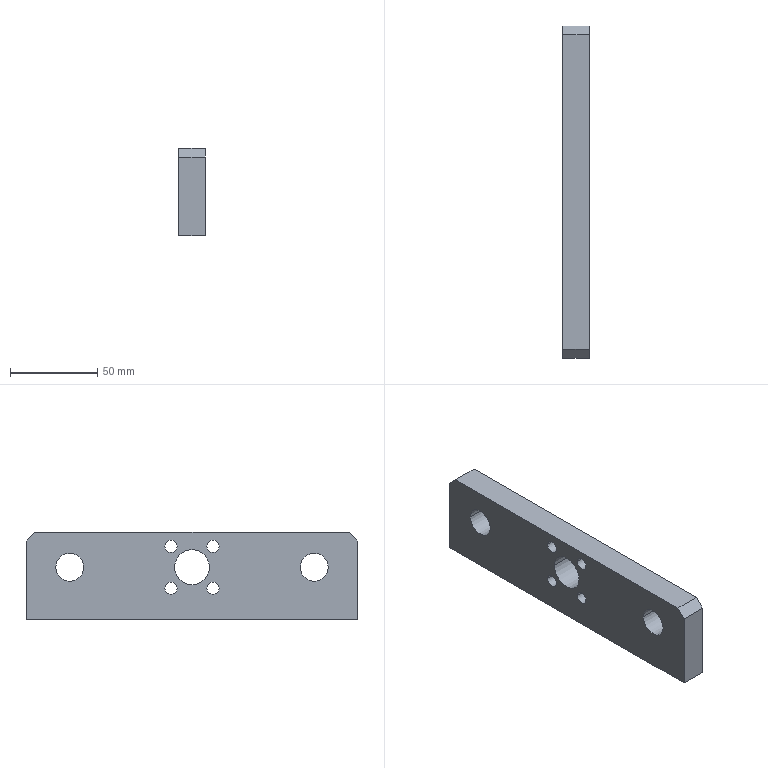Component | SolidWorks | DoubleFilmTransport-1_SupportPlate-1 | 1 solid | 46 faces | box 15 x 190 x 50 mm | volume 124028 mm3 | cylinder 26 | plane 12 | cone 8 | commonest cylinder face diameters 11 x8 7 x8 8.5 x4 16 x4 20 x2
build123d program:
from build123d import *

# Parameters (mm, degrees)
SKETCH1_W                                            = 190
SKETCH1_H                                            = 50
BOSS_EXTRUDE1_DEPTH                                  = 15
F_20_0_20_DIAMETER_HOLE1_D                           = 20
F_16_0_16_DIAMETER_HOLE1_D                           = 16
CYLINDRICAL_COUNTERSUNK_HOLE_1_FOR_M6_HE_D           = 7
CYLINDRICAL_COUNTERSUNK_HOLE_1_FOR_M6_HE_CBORE_D     = 11
CYLINDRICAL_COUNTERSUNK_HOLE_1_FOR_M6_HE_CBORE_DEPTH = 8
F_8_5_8_5_DIAMETER_HOLE1_D                           = 8.5
F_8_5_8_5_DIAMETER_HOLE1_DEPTH                       = 27.5
F_8_5_8_5_DIAMETER_HOLE1_TIP                         = 2.554
CHAMFER1_SIZE                                        = 0.775
CHAMFER2_SIZE                                        = 5


with BuildPart() as part:
    # Sketch1 → Boss-Extrude1 (new body)
    with BuildSketch(Plane.XY.offset(7.5)):
        with Locations((0, 25)):
            Rectangle(SKETCH1_W, SKETCH1_H)
    extrude(amount=-BOSS_EXTRUDE1_DEPTH)

    # 20.0 _20_ Diameter Hole1 (through all)
    with Locations(Plane(origin=(0, 0, -7.5), x_dir=(-1, 0, 0), z_dir=(0, 0, -1))):
        with Locations((0, 30)):
            Hole(F_20_0_20_DIAMETER_HOLE1_D / 2)

    # 16.0 _16_ Diameter Hole1 (through all)
    with Locations(Plane(origin=(0, 0, -7.5), x_dir=(-1, 0, 0), z_dir=(0, 0, -1))):
        with Locations((-70, 30), (70, 30)):
            Hole(F_16_0_16_DIAMETER_HOLE1_D / 2)

    # Cylindrical Countersunk Hole 1 for M6 He (through all)
    with Locations(Plane.XY.offset(7.5)):
        with Locations((-12, 42), (-12, 18), (12, 42), (12, 18)):
            CounterBoreHole(CYLINDRICAL_COUNTERSUNK_HOLE_1_FOR_M6_HE_D / 2, CYLINDRICAL_COUNTERSUNK_HOLE_1_FOR_M6_HE_CBORE_D / 2, CYLINDRICAL_COUNTERSUNK_HOLE_1_FOR_M6_HE_CBORE_DEPTH)

    # 8.5 _8.5_ Diameter Hole1
    with Locations(Plane(origin=(0, 0, 0), x_dir=(-1, 0, 0), z_dir=(0, -1, 0))):
        with Locations((-50, 0), (50, 0)):
            Hole(F_8_5_8_5_DIAMETER_HOLE1_D / 2, depth=F_8_5_8_5_DIAMETER_HOLE1_DEPTH)
            with Locations((0, 0, -(F_8_5_8_5_DIAMETER_HOLE1_DEPTH + F_8_5_8_5_DIAMETER_HOLE1_TIP / 2))):  # 118° drill point
                Cone(0, F_8_5_8_5_DIAMETER_HOLE1_D / 2, F_8_5_8_5_DIAMETER_HOLE1_TIP, mode=Mode.SUBTRACT)

    # Chamfer1
    chamfer1_edges = [part.edges().sort_by_distance(p)[0] for p in [
        (-54.25, 0, 0),
        (45.75, 0, 0),
    ]]
    chamfer(chamfer1_edges, length=CHAMFER1_SIZE)

    # Chamfer2
    chamfer2_edges = [part.edges().sort_by_distance(p)[0] for p in [
        (-95, 50, 0),
        (95, 50, 0),
    ]]
    chamfer(chamfer2_edges, length=CHAMFER2_SIZE)


solid = part.part

# Placed as in the assembly
solid = solid.moved(Location((-457.746, 115.373, -16.5), (90, 90, 0)))